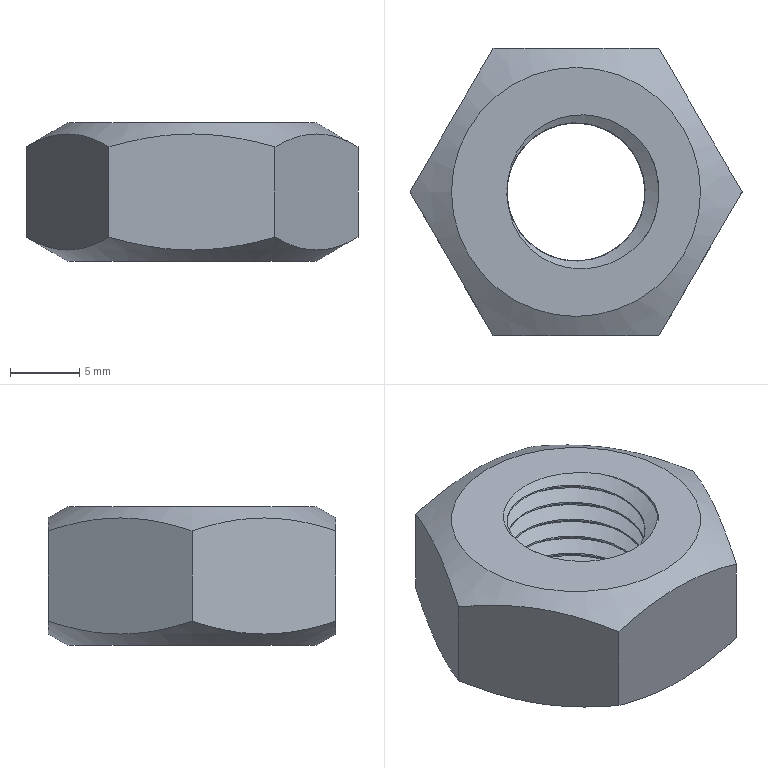Component | NX | NUT_M10 | 1 solid | 15 faces | volume 2637 mm3 | plane 9 | cylinder 2 | spline 2 | cone 2 | commonest cylinder face diameters 10 x1 12 x1